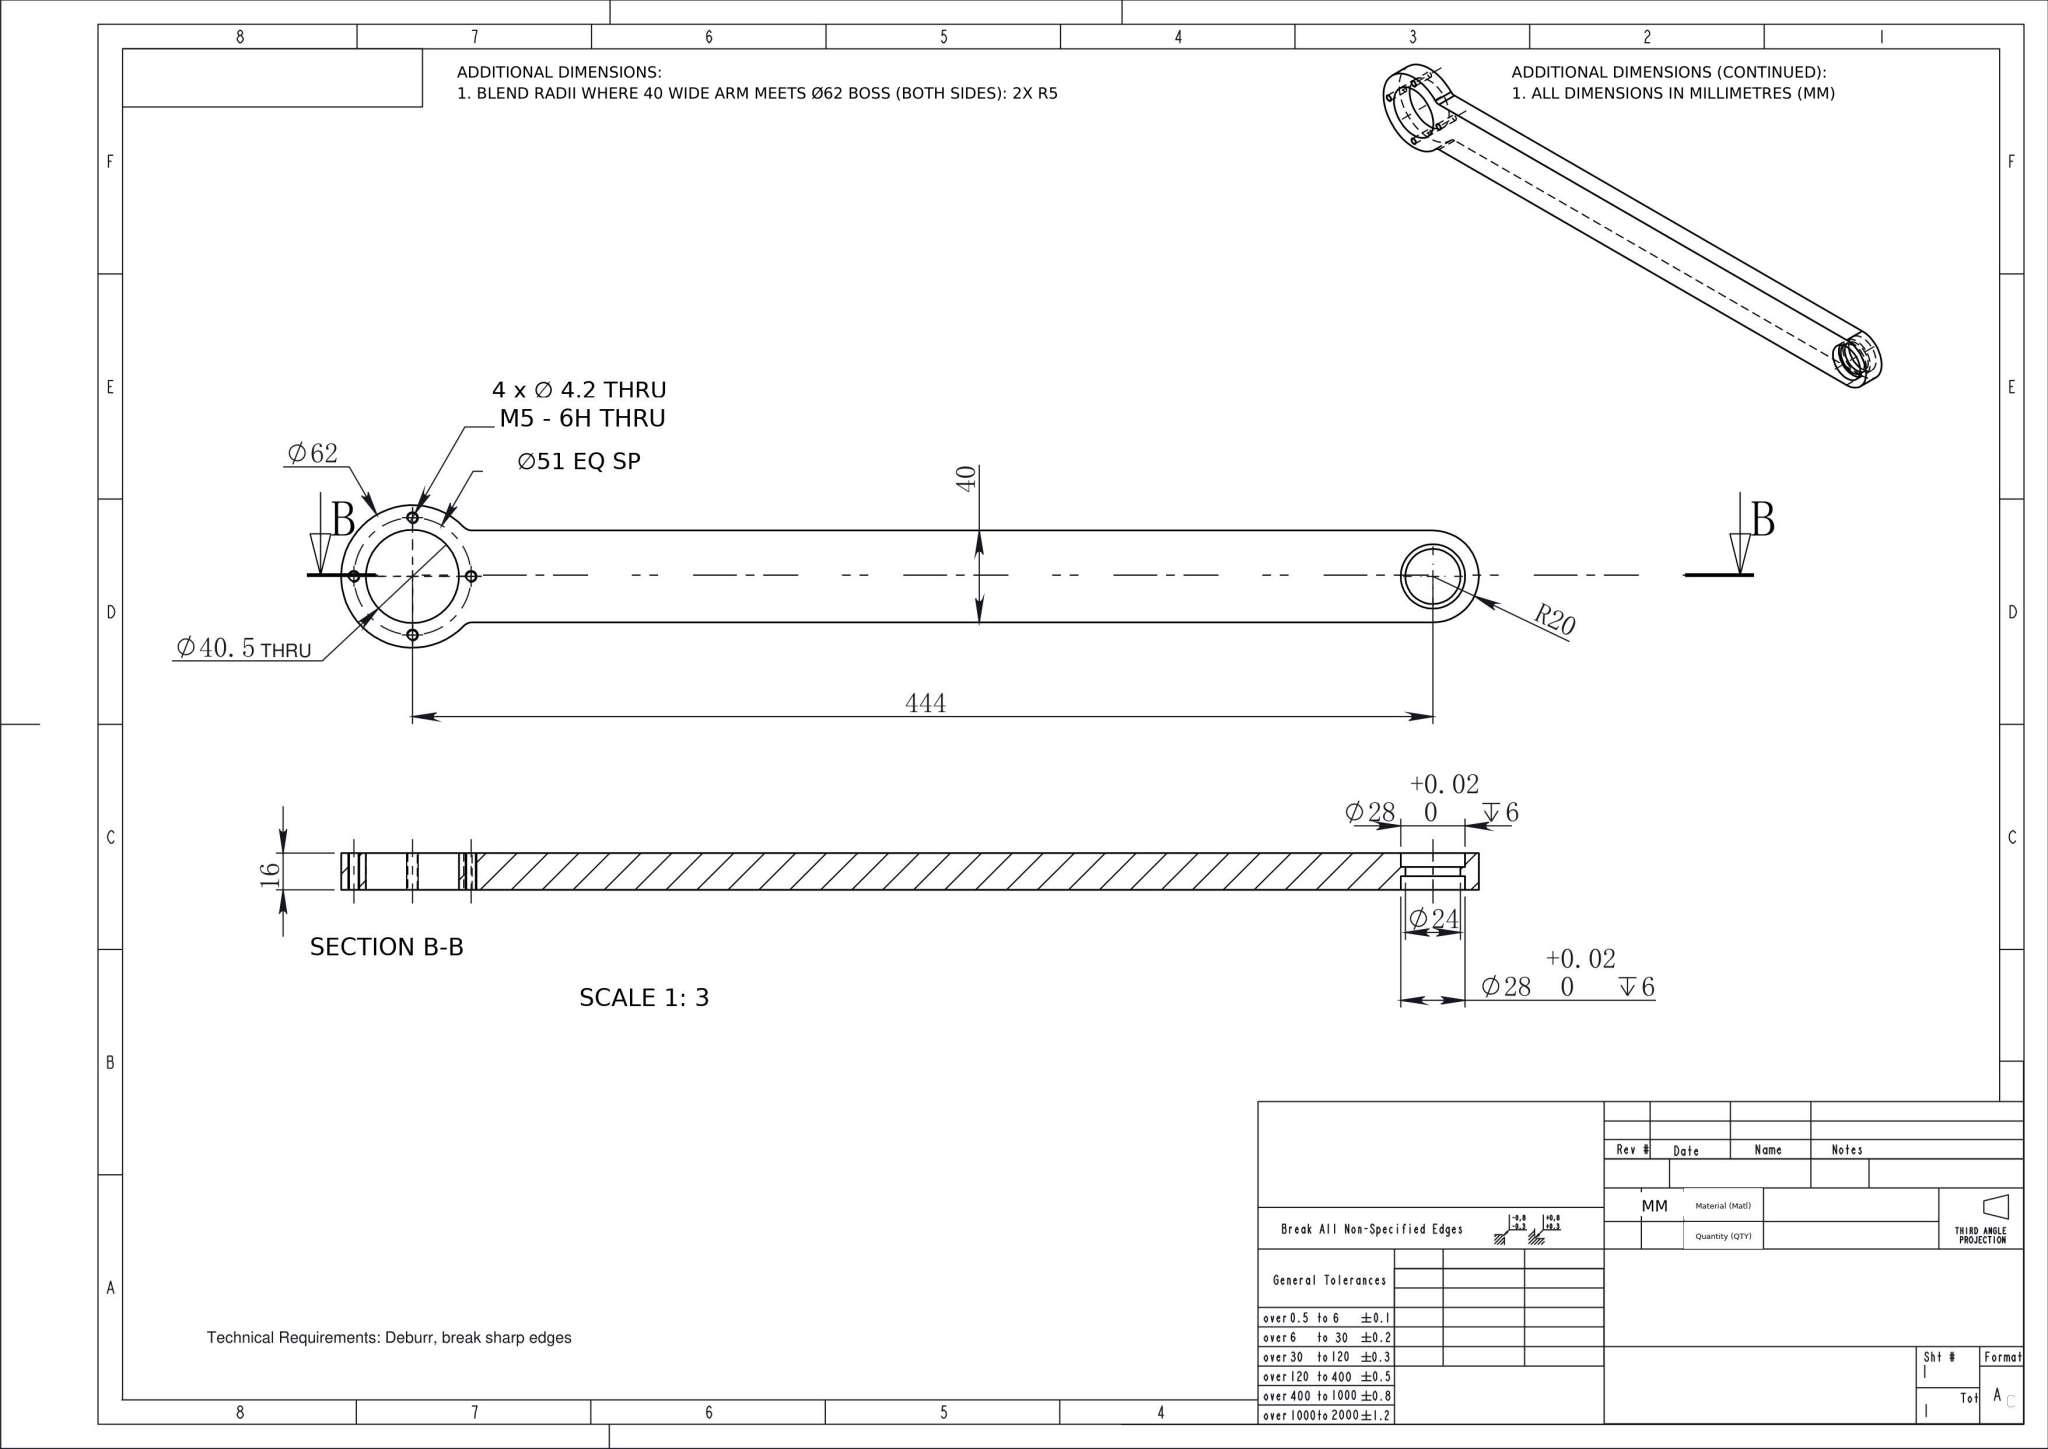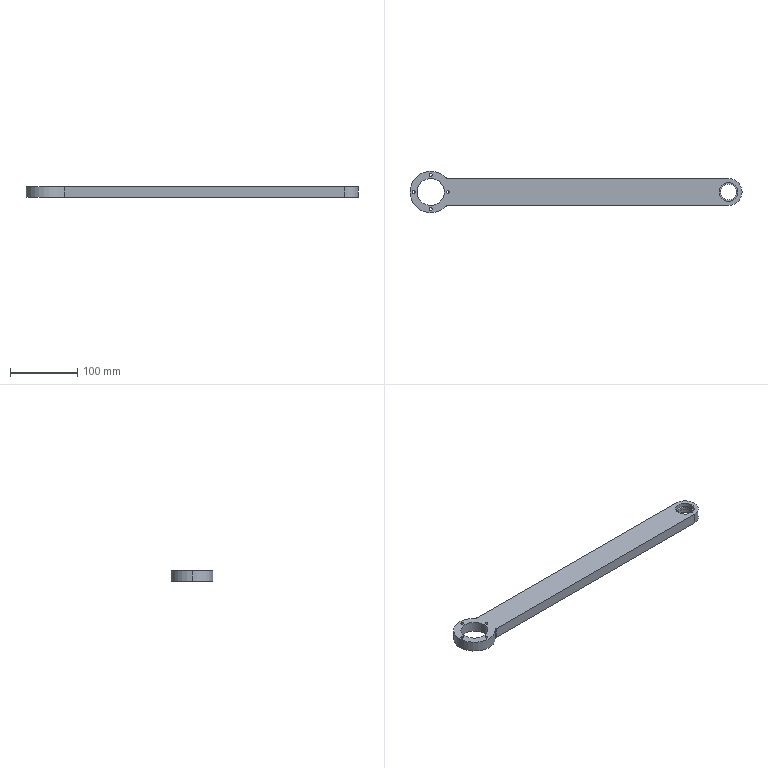Part | NX | mm | 1 solid | 28 faces | box 495 x 62 x 16 mm | volume 293479 mm3 | cylinder 22 | plane 6 | commonest cylinder face diameters 4.2 x8 28 x4 40 x2 62 x2 40.5 x2 24 x2 10 x2